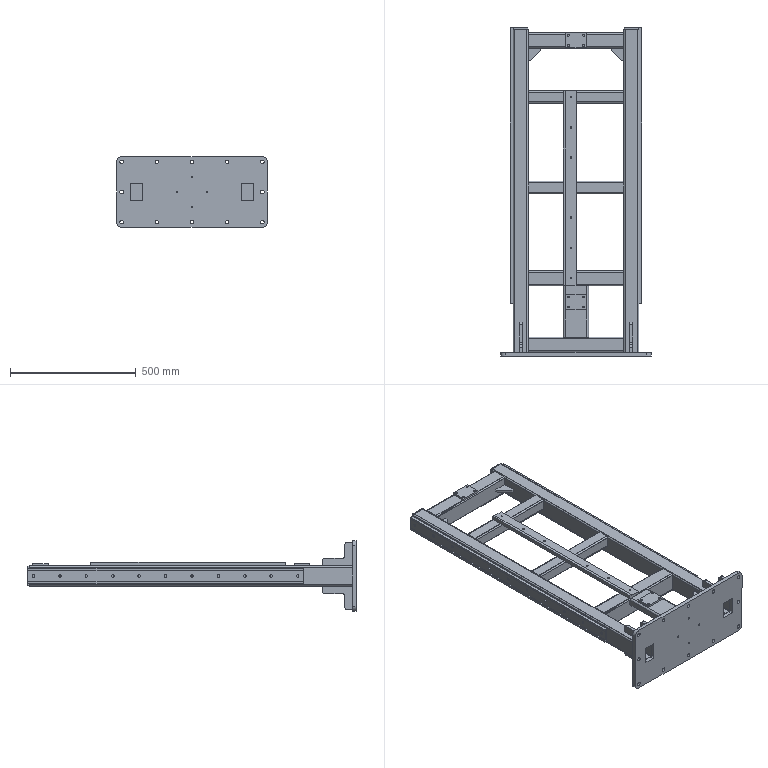Component | SolidWorks | UprightFrame-1 | 22 solids | 468 faces | volume 7765426 mm3 | cylinder 268 | plane 200 | commonest cylinder face diameters 10.2 x88 6.8 x60 14 x26 12 x20 6 x20 20 x12 12.8 x8 6.4 x8